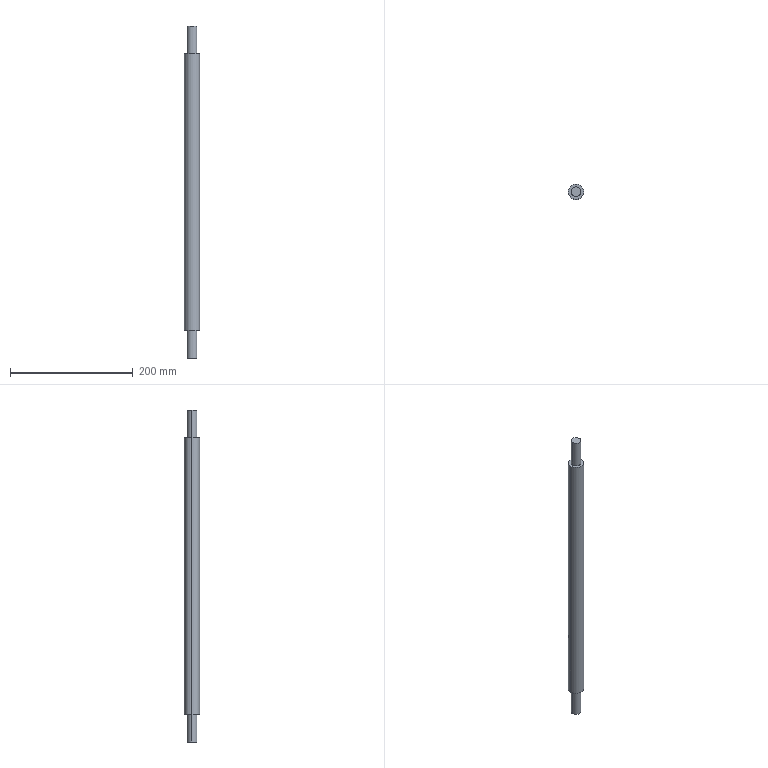Component | SolidWorks | GuidePostXG-XG1-1 | 1 solid | 10 faces | box 25 x 25 x 540 mm | volume 238989 mm3 | cylinder 6 | plane 4 | commonest cylinder face diameters 16 x4 25 x2
build123d program:
from build123d import *


with BuildPart() as part:
    # Sketch1 → Revolve1 (revolve)
    with BuildSketch(Plane(origin=(0, 0, 0), x_dir=(1, 0, 0), z_dir=(0, 1, 0)), mode=Mode.PRIVATE) as revolve1_sk:
        Polygon((0, 0), (0, 8), (45, 8), (45, 12.5), (495, 12.5), (495, 8), (540, 8), (540, 0), align=None)
    revolve(revolve1_sk.sketch.rotate(Axis((-2616.332, 0, 0), (1, 0, 0)), 180), axis=Axis((-2616.332, 0, 0), (1, 0, 0)))


solid = part.part

# Placed as in the assembly
solid = solid.moved(Location((-348.72, 545, 313), (0, 90, 0)))
STEP:
#1=COLOUR_RGB('',0.7922,0.8196,0.9333);
#2=FILL_AREA_STYLE_COLOUR('',#1);
#3=FILL_AREA_STYLE('',(#2));
#4=SURFACE_STYLE_FILL_AREA(#3);
#5=SURFACE_SIDE_STYLE('',(#4));
#6=SURFACE_STYLE_USAGE(.BOTH.,#5);
#7=PRESENTATION_STYLE_ASSIGNMENT((#6));
#8=CARTESIAN_POINT('',(-13.414,21.457,-8.937));
#9=VERTEX_POINT('',#8);
#10=CARTESIAN_POINT('',(-14.044,21.457,-8.937));
#11=VERTEX_POINT('',#10);
#12=CARTESIAN_POINT('',(-13.729,21.457,-8.937));
#13=DIRECTION('',(0.,-0.,1.));
#14=DIRECTION('',(1.,-0.0001876,0.));
#15=AXIS2_PLACEMENT_3D('',#12,#13,#14);
#16=CIRCLE('',#15,0.315);
#17=EDGE_CURVE('',#9,#11,#16,.T.);
#18=ORIENTED_EDGE('',*,*,#17,.T.);
#19=CARTESIAN_POINT('',(-14.044,21.457,-7.165));
#20=VERTEX_POINT('',#19);
#21=CARTESIAN_POINT('',(-14.044,21.457,115.328));
#22=DIRECTION('',(0.,-0.,1.));
#23=VECTOR('',#22,39.37);
#24=LINE('',#21,#23);
#25=EDGE_CURVE('',#11,#20,#24,.T.);
#26=ORIENTED_EDGE('',*,*,#25,.T.);
#27=CARTESIAN_POINT('',(-13.414,21.457,-7.165));
#28=VERTEX_POINT('',#27);
#29=CARTESIAN_POINT('',(-13.729,21.457,-7.165));
#30=DIRECTION('',(0.,-0.,1.));
#31=DIRECTION('',(1.,-0.0001876,0.));
#32=AXIS2_PLACEMENT_3D('',#29,#30,#31);
#33=CIRCLE('',#32,0.315);
#34=EDGE_CURVE('',#28,#20,#33,.T.);
#35=ORIENTED_EDGE('',*,*,#34,.F.);
#36=CARTESIAN_POINT('',(-13.414,21.457,115.328));
#37=DIRECTION('',(0.,-0.,1.));
#38=VECTOR('',#37,39.37);
#39=LINE('',#36,#38);
#40=EDGE_CURVE('',#9,#28,#39,.T.);
#41=ORIENTED_EDGE('',*,*,#40,.F.);
#42=EDGE_LOOP('',(#18,#26,#35,#41));
#43=FACE_OUTER_BOUND('',#42,.T.);
#44=CARTESIAN_POINT('',(-13.729,21.457,115.328));
#45=DIRECTION('',(0.,-0.,1.));
#46=DIRECTION('',(1.,-0.0001876,0.));
#47=AXIS2_PLACEMENT_3D('',#44,#45,#46);
#48=CYLINDRICAL_SURFACE('',#47,0.315);
#49=ADVANCED_FACE('',(#43),#48,.T.);
#50=CARTESIAN_POINT('',(-13.237,21.457,-7.165));
#51=VERTEX_POINT('',#50);
#52=CARTESIAN_POINT('',(-14.221,21.457,-7.165));
#53=VERTEX_POINT('',#52);
#54=CARTESIAN_POINT('',(-13.729,21.457,-7.165));
#55=DIRECTION('',(0.,-0.,1.));
#56=DIRECTION('',(1.,-0.0001876,0.));
#57=AXIS2_PLACEMENT_3D('',#54,#55,#56);
#58=CIRCLE('',#57,0.4921);
#59=EDGE_CURVE('',#51,#53,#58,.T.);
#60=ORIENTED_EDGE('',*,*,#59,.T.);
#61=CARTESIAN_POINT('',(-14.221,21.457,10.551));
#62=VERTEX_POINT('',#61);
#63=CARTESIAN_POINT('',(-14.221,21.457,115.328));
#64=DIRECTION('',(0.,-0.,1.));
#65=VECTOR('',#64,39.37);
#66=LINE('',#63,#65);
#67=EDGE_CURVE('',#53,#62,#66,.T.);
#68=ORIENTED_EDGE('',*,*,#67,.T.);
#69=CARTESIAN_POINT('',(-13.237,21.457,10.551));
#70=VERTEX_POINT('',#69);
#71=CARTESIAN_POINT('',(-13.729,21.457,10.551));
#72=DIRECTION('',(0.,-0.,1.));
#73=DIRECTION('',(1.,-0.0001876,0.));
#74=AXIS2_PLACEMENT_3D('',#71,#72,#73);
#75=CIRCLE('',#74,0.4921);
#76=EDGE_CURVE('',#70,#62,#75,.T.);
#77=ORIENTED_EDGE('',*,*,#76,.F.);
#78=CARTESIAN_POINT('',(-13.237,21.457,115.328));
#79=DIRECTION('',(0.,-0.,1.));
#80=VECTOR('',#79,39.37);
#81=LINE('',#78,#80);
#82=EDGE_CURVE('',#51,#70,#81,.T.);
#83=ORIENTED_EDGE('',*,*,#82,.F.);
#84=EDGE_LOOP('',(#60,#68,#77,#83));
#85=FACE_OUTER_BOUND('',#84,.T.);
#86=CARTESIAN_POINT('',(-13.729,21.457,115.328));
#87=DIRECTION('',(0.,-0.,1.));
#88=DIRECTION('',(1.,-0.0001876,0.));
#89=AXIS2_PLACEMENT_3D('',#86,#87,#88);
#90=CYLINDRICAL_SURFACE('',#89,0.4921);
#91=ADVANCED_FACE('',(#85),#90,.T.);
#92=CARTESIAN_POINT('',(-13.414,21.457,10.551));
#93=VERTEX_POINT('',#92);
#94=CARTESIAN_POINT('',(-14.044,21.457,10.551));
#95=VERTEX_POINT('',#94);
#96=CARTESIAN_POINT('',(-13.729,21.457,10.551));
#97=DIRECTION('',(0.,-0.,1.));
#98=DIRECTION('',(1.,-0.0001876,0.));
#99=AXIS2_PLACEMENT_3D('',#96,#97,#98);
#100=CIRCLE('',#99,0.315);
#101=EDGE_CURVE('',#93,#95,#100,.T.);
#102=ORIENTED_EDGE('',*,*,#101,.T.);
#103=CARTESIAN_POINT('',(-14.044,21.457,12.323));
#104=VERTEX_POINT('',#103);
#105=CARTESIAN_POINT('',(-14.044,21.457,115.328));
#106=DIRECTION('',(0.,-0.,1.));
#107=VECTOR('',#106,39.37);
#108=LINE('',#105,#107);
#109=EDGE_CURVE('',#95,#104,#108,.T.);
#110=ORIENTED_EDGE('',*,*,#109,.T.);
#111=CARTESIAN_POINT('',(-13.414,21.457,12.323));
#112=VERTEX_POINT('',#111);
#113=CARTESIAN_POINT('',(-13.729,21.457,12.323));
#114=DIRECTION('',(0.,-0.,1.));
#115=DIRECTION('',(1.,-0.0001876,0.));
#116=AXIS2_PLACEMENT_3D('',#113,#114,#115);
#117=CIRCLE('',#116,0.315);
#118=EDGE_CURVE('',#112,#104,#117,.T.);
#119=ORIENTED_EDGE('',*,*,#118,.F.);
#120=CARTESIAN_POINT('',(-13.414,21.457,115.328));
#121=DIRECTION('',(0.,-0.,1.));
#122=VECTOR('',#121,39.37);
#123=LINE('',#120,#122);
#124=EDGE_CURVE('',#93,#112,#123,.T.);
#125=ORIENTED_EDGE('',*,*,#124,.F.);
#126=EDGE_LOOP('',(#102,#110,#119,#125));
#127=FACE_OUTER_BOUND('',#126,.T.);
#128=CARTESIAN_POINT('',(-13.729,21.457,115.328));
#129=DIRECTION('',(0.,-0.,1.));
#130=DIRECTION('',(1.,-0.0001876,0.));
#131=AXIS2_PLACEMENT_3D('',#128,#129,#130);
#132=CYLINDRICAL_SURFACE('',#131,0.315);
#133=ADVANCED_FACE('',(#127),#132,.T.);
#134=ORIENTED_EDGE('',*,*,#118,.T.);
#135=CARTESIAN_POINT('',(-13.729,21.457,12.323));
#136=DIRECTION('',(0.,-0.,1.));
#137=DIRECTION('',(1.,-0.0001876,0.));
#138=AXIS2_PLACEMENT_3D('',#135,#136,#137);
#139=CIRCLE('',#138,0.315);
#140=EDGE_CURVE('',#104,#112,#139,.T.);
#141=ORIENTED_EDGE('',*,*,#140,.T.);
#142=EDGE_LOOP('',(#134,#141));
#143=FACE_OUTER_BOUND('',#142,.T.);
#144=CARTESIAN_POINT('',(-13.729,21.457,12.323));
#145=DIRECTION('',(-0.,0.,-1.));
#146=DIRECTION('',(-1.,0.0001876,0.));
#147=AXIS2_PLACEMENT_3D('',#144,#145,#146);
#148=PLANE('',#147);
#149=ADVANCED_FACE('',(#143),#148,.F.);
#150=ORIENTED_EDGE('',*,*,#109,.F.);
#151=CARTESIAN_POINT('',(-13.729,21.457,10.551));
#152=DIRECTION('',(0.,-0.,1.));
#153=DIRECTION('',(1.,-0.0001876,0.));
#154=AXIS2_PLACEMENT_3D('',#151,#152,#153);
#155=CIRCLE('',#154,0.315);
#156=EDGE_CURVE('',#95,#93,#155,.T.);
#157=ORIENTED_EDGE('',*,*,#156,.T.);
#158=ORIENTED_EDGE('',*,*,#124,.T.);
#159=ORIENTED_EDGE('',*,*,#140,.F.);
#160=EDGE_LOOP('',(#150,#157,#158,#159));
#161=FACE_OUTER_BOUND('',#160,.T.);
#162=CARTESIAN_POINT('',(-13.729,21.457,115.328));
#163=DIRECTION('',(0.,-0.,1.));
#164=DIRECTION('',(1.,-0.0001876,0.));
#165=AXIS2_PLACEMENT_3D('',#162,#163,#164);
#166=CYLINDRICAL_SURFACE('',#165,0.315);
#167=ADVANCED_FACE('',(#161),#166,.T.);
#168=ORIENTED_EDGE('',*,*,#101,.F.);
#169=ORIENTED_EDGE('',*,*,#156,.F.);
#170=EDGE_LOOP('',(#168,#169));
#171=FACE_BOUND('',#170,.T.);
#172=ORIENTED_EDGE('',*,*,#76,.T.);
#173=CARTESIAN_POINT('',(-13.729,21.457,10.551));
#174=DIRECTION('',(0.,-0.,1.));
#175=DIRECTION('',(1.,-0.0001876,0.));
#176=AXIS2_PLACEMENT_3D('',#173,#174,#175);
#177=CIRCLE('',#176,0.4921);
#178=EDGE_CURVE('',#62,#70,#177,.T.);
#179=ORIENTED_EDGE('',*,*,#178,.T.);
#180=EDGE_LOOP('',(#172,#179));
#181=FACE_OUTER_BOUND('',#180,.T.);
#182=CARTESIAN_POINT('',(-14.044,21.457,10.551));
#183=DIRECTION('',(-0.,0.,-1.));
#184=DIRECTION('',(-1.,0.0001876,0.));
#185=AXIS2_PLACEMENT_3D('',#182,#183,#184);
#186=PLANE('',#185);
#187=ADVANCED_FACE('',(#171,#181),#186,.F.);
#188=ORIENTED_EDGE('',*,*,#67,.F.);
#189=CARTESIAN_POINT('',(-13.729,21.457,-7.165));
#190=DIRECTION('',(0.,-0.,1.));
#191=DIRECTION('',(1.,-0.0001876,0.));
#192=AXIS2_PLACEMENT_3D('',#189,#190,#191);
#193=CIRCLE('',#192,0.4921);
#194=EDGE_CURVE('',#53,#51,#193,.T.);
#195=ORIENTED_EDGE('',*,*,#194,.T.);
#196=ORIENTED_EDGE('',*,*,#82,.T.);
#197=ORIENTED_EDGE('',*,*,#178,.F.);
#198=EDGE_LOOP('',(#188,#195,#196,#197));
#199=FACE_OUTER_BOUND('',#198,.T.);
#200=CARTESIAN_POINT('',(-13.729,21.457,115.328));
#201=DIRECTION('',(0.,-0.,1.));
#202=DIRECTION('',(1.,-0.0001876,0.));
#203=AXIS2_PLACEMENT_3D('',#200,#201,#202);
#204=CYLINDRICAL_SURFACE('',#203,0.4921);
#205=ADVANCED_FACE('',(#199),#204,.T.);
#206=ORIENTED_EDGE('',*,*,#59,.F.);
#207=ORIENTED_EDGE('',*,*,#194,.F.);
#208=EDGE_LOOP('',(#206,#207));
#209=FACE_OUTER_BOUND('',#208,.T.);
#210=ORIENTED_EDGE('',*,*,#34,.T.);
#211=CARTESIAN_POINT('',(-13.729,21.457,-7.165));
#212=DIRECTION('',(0.,-0.,1.));
#213=DIRECTION('',(1.,-0.0001876,0.));
#214=AXIS2_PLACEMENT_3D('',#211,#212,#213);
#215=CIRCLE('',#214,0.315);
#216=EDGE_CURVE('',#20,#28,#215,.T.);
#217=ORIENTED_EDGE('',*,*,#216,.T.);
#218=EDGE_LOOP('',(#210,#217));
#219=FACE_BOUND('',#218,.T.);
#220=CARTESIAN_POINT('',(-14.221,21.457,-7.165));
#221=DIRECTION('',(0.,-0.,1.));
#222=DIRECTION('',(1.,-0.0001876,-0.));
#223=AXIS2_PLACEMENT_3D('',#220,#221,#222);
#224=PLANE('',#223);
#225=ADVANCED_FACE('',(#209,#219),#224,.F.);
#226=ORIENTED_EDGE('',*,*,#25,.F.);
#227=CARTESIAN_POINT('',(-13.729,21.457,-8.937));
#228=DIRECTION('',(0.,-0.,1.));
#229=DIRECTION('',(1.,-0.0001876,0.));
#230=AXIS2_PLACEMENT_3D('',#227,#228,#229);
#231=CIRCLE('',#230,0.315);
#232=EDGE_CURVE('',#11,#9,#231,.T.);
#233=ORIENTED_EDGE('',*,*,#232,.T.);
#234=ORIENTED_EDGE('',*,*,#40,.T.);
#235=ORIENTED_EDGE('',*,*,#216,.F.);
#236=EDGE_LOOP('',(#226,#233,#234,#235));
#237=FACE_OUTER_BOUND('',#236,.T.);
#238=CARTESIAN_POINT('',(-13.729,21.457,115.328));
#239=DIRECTION('',(0.,-0.,1.));
#240=DIRECTION('',(1.,-0.0001876,0.));
#241=AXIS2_PLACEMENT_3D('',#238,#239,#240);
#242=CYLINDRICAL_SURFACE('',#241,0.315);
#243=ADVANCED_FACE('',(#237),#242,.T.);
#244=ORIENTED_EDGE('',*,*,#17,.F.);
#245=ORIENTED_EDGE('',*,*,#232,.F.);
#246=EDGE_LOOP('',(#244,#245));
#247=FACE_OUTER_BOUND('',#246,.T.);
#248=CARTESIAN_POINT('',(-14.044,21.457,-8.937));
#249=DIRECTION('',(0.,-0.,1.));
#250=DIRECTION('',(1.,-0.0001876,-0.));
#251=AXIS2_PLACEMENT_3D('',#248,#249,#250);
#252=PLANE('',#251);
#253=ADVANCED_FACE('',(#247),#252,.F.);
#254=CLOSED_SHELL('',(#49,#91,#133,#149,#167,#187,#205,#225,#243,#253));
#255=MANIFOLD_SOLID_BREP('',#254);
#256=STYLED_ITEM('',(#7),#255);
#257=(LENGTH_UNIT()NAMED_UNIT(*)SI_UNIT($,.METRE.));
#258=LENGTH_MEASURE_WITH_UNIT(LENGTH_MEASURE(0.0254),#257);
#259=DIMENSIONAL_EXPONENTS(1.,0.,0.,0.,0.,0.,0.);
#260=(CONVERSION_BASED_UNIT('',#258)LENGTH_UNIT()NAMED_UNIT(#259));
#261=UNCERTAINTY_MEASURE_WITH_UNIT(LENGTH_MEASURE(0.00001),#260,'','');
#262=(NAMED_UNIT(*)PLANE_ANGLE_UNIT()SI_UNIT($,.RADIAN.));
#263=(NAMED_UNIT(*)SI_UNIT($,.STERADIAN.)SOLID_ANGLE_UNIT());
#264=(GEOMETRIC_REPRESENTATION_CONTEXT(3)GLOBAL_UNCERTAINTY_ASSIGNED_CONTEXT((#261))GLOBAL_UNIT_ASSIGNED_CONTEXT((#260,#262,#263))REPRESENTATION_CONTEXT('',''));
#265=MECHANICAL_DESIGN_GEOMETRIC_PRESENTATION_REPRESENTATION('',(#256),#264);
#266=PRESENTATION_LAYER_ASSIGNMENT('','',(#256));
#267=CARTESIAN_POINT('',(0.,0.,0.));
#268=DIRECTION('',(0.,0.,1.));
#269=DIRECTION('',(1.,0.,0.));
#270=AXIS2_PLACEMENT_3D('',#267,#268,#269);
#271=(LENGTH_UNIT()NAMED_UNIT(*)SI_UNIT($,.METRE.));
#272=LENGTH_MEASURE_WITH_UNIT(LENGTH_MEASURE(0.0254),#271);
#273=DIMENSIONAL_EXPONENTS(1.,0.,0.,0.,0.,0.,0.);
#274=(CONVERSION_BASED_UNIT('',#272)LENGTH_UNIT()NAMED_UNIT(#273));
#275=UNCERTAINTY_MEASURE_WITH_UNIT(LENGTH_MEASURE(0.00001),#274,'','');
#276=(NAMED_UNIT(*)PLANE_ANGLE_UNIT()SI_UNIT($,.RADIAN.));
#277=(NAMED_UNIT(*)SI_UNIT($,.STERADIAN.)SOLID_ANGLE_UNIT());
#278=(GEOMETRIC_REPRESENTATION_CONTEXT(3)GLOBAL_UNCERTAINTY_ASSIGNED_CONTEXT((#275))GLOBAL_UNIT_ASSIGNED_CONTEXT((#274,#276,#277))REPRESENTATION_CONTEXT('',''));
#279=ADVANCED_BREP_SHAPE_REPRESENTATION('',(#255,#270),#278);